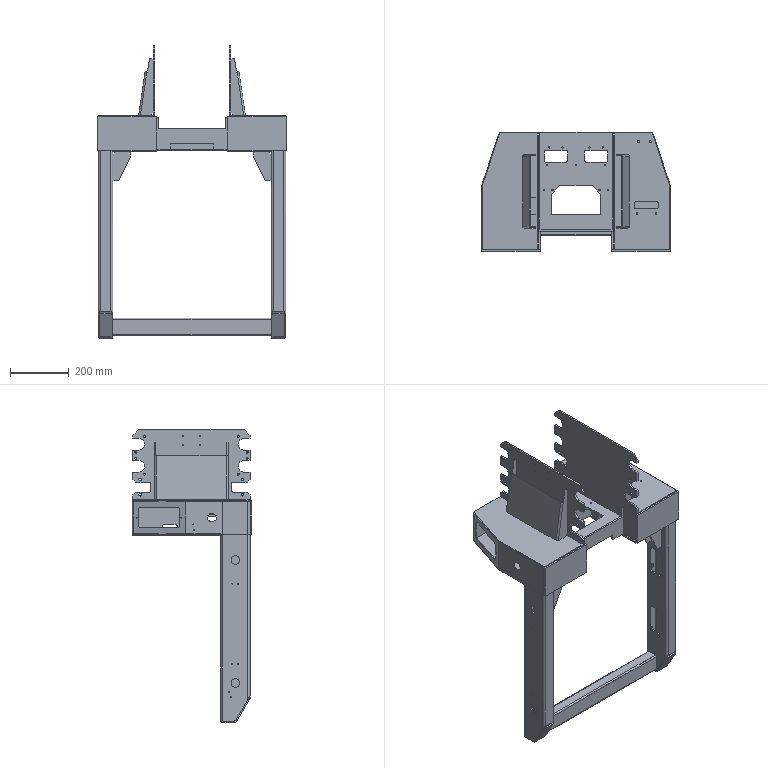Assembly | SolidWorks | mm | 23 component files | 23 solids | 730 faces | box 644 x 408 x 999 mm | volume 6835255 mm3 | plane 404 | cylinder 326 | commonest cylinder face diameters 3.3 x48 4.2 x46 20 x44 10 x37 6.8 x36 5 x20 9 x16 8 x16
Bill of materials:
JHK-B1001LeftRectangularTubeBeam | 1 | Q235A | Straight hollow rectangular tube with rounded corners. One end is cut at an angle across part of the section, and one wide face has two small features spaced along its length.
JHK-B1002RightRectangularTubeBeam | 1 | Q235A | Straight hollow rectangular tube with rounded corners and an angled cut at one end. One face has two round holes spaced along its length, plus a few very small marks.
JHK-B1003RightRearBaffle | 1 | Q235A | Flat plate of constant thickness, outline rectangular except for one long diagonal edge that trims a corner. It has a rounded-rectangle through slot and four small round holes.
JHK-B1004Stiffener | 4 | Q235A | Solid block extruded from a constant-thickness irregular quadrilateral profile: one straight vertical edge, a short chamfer at one top corner, and a long inclined edge that tapers the shape toward the bottom.
THK-B1001RollerBracketLeft | 1 | Q235A | Thin flat plate with a near-symmetric outline: chamfered top corners, two rounded U-shaped slots and one rectangular notch on each side edge, and rectangular notches plus a narrow slit along the bottom edge. It has multiple round holes, including a four-hole pattern near the top center.
THK-B1002RollerBracketRight | 1 | Q235A | Thin flat plate with chamfered top corners, paired U-shaped side slots, rectangular side notches, bottom-edge rectangular notches and a slit, and multiple round holes.
THK-B1003LeftRearBaffle | 1 | Q235A | Flat plate of constant thickness with one long diagonal edge trimming a corner and a single rounded-rectangle notch cut into one straight edge. No holes.
THK-B1005LeftFrontBaffle | 1 | Q235A | Flat plate of constant thickness with one long diagonal edge, a stepped rectangular cutout at one corner (L-shaped outline), and two small round holes along the straight edge.
THK-B1006RightFrontBaffle | 1 | Q235A | Flat plate of constant thickness with one long diagonal edge, a stepped rectangular corner cutout, a rounded-square through opening, two tiny holes above the opening, and two small holes along the straight edge.
THK-B1009MiddleSpacer | 1 | Q235A | Rectangular flat plate with small corner chamfers. It has two rounded-rectangle through openings, one large opening with chamfered upper corners, and many small round holes.
THK-B1011LooseRopeProtectionMountingPlate | 1 | Q235A | Rectangular flat bar with chamfered corners and two round through holes side by side near the center.
THK-B1012LowerBaffle | 1 | Q235A | Flat plate of constant thickness shaped as a long strip. Two narrow rectangular tabs project from the top edge near each end, and a wide shallow rectangular relief is cut into the middle of the bottom edge.
THK-B1013LowerSupportPlate | 2 | Q235A | Thin flat rectangular plate with uniform thickness and square edges; no holes or cutouts are visible.
THK-B1014SideStiffenerPlate | 2 | Q235A | Channel-shaped (C-section) formed part with a wide flat web and two side flanges joined by rounded bends. The flanges are tapered, so they are trapezoidal in side view, and they stick up past the web edge as narrow tabs. One bottom corner of each flange has a chamfer.
THK-B1015RectangularTubeEndSealingPlate | 2 | Q235A | Bent flat strip forming an angle shape: one longer leg slanted at an obtuse angle to a shorter flat leg, joined by a single rounded bend. The free-end corners are rounded and the thickness is uniform.
THK-B1016UpperCoverPlate | 1 | Q235A | Thin-wall formed band bracket, open at one side. It has a straight center segment, two angled segments and two parallel end legs. The top edge of the center segment has a wide rectangular notch. Each angled segment has a large rounded-rectangle cutout with small holes on either side of it. Each end leg has one round hole and a pair of small holes.
THK-B1017FrontCrossBeam | 1 | Q235A | Straight hollow rectangular tube with rounded outer and inner corners and constant wall thickness. Both ends are cut square and no holes are visible along its length.
Mates:
1. coincident | THK-B1003LeftRearBaffle-1 face at (-133, 200, -145) dir (0, 1, 0) | THK-B1005LeftFrontBaffle-1 face at (-260, 200, -255) dir (0, 1, 0)
2. coincident | JHK-B1003RightRearBaffle-1 face at (133, 200, -145) dir (0, 1, 0) | THK-B1006RightFrontBaffle-1 face at (122, 200, -255) dir (0, 1, 0)
3. coincident | THK-B1003LeftRearBaffle-1 face at (-133, 200, -145) dir (0, 1, 0) | JHK-B1003RightRearBaffle-1 face at (133, 200, -145) dir (0, 1, 0)
4. coincident | THK-B1003LeftRearBaffle-1 face at (-133, 200, -145) dir (0, 1, 0) | THK-B1016UpperCoverPlate-1 face at (-260, 200, -142) dir (0, -1, 0)
5. coincident | JHK-B1001LeftRectangularTubeBeam-1 plane at (-295, -150, -520) dir (0, 1, 0) | JHK-B1002RightRectangularTubeBeam-1 plane at (295, -150, -520) dir (0, 1, 0)
6. coincident | JHK-B1001LeftRectangularTubeBeam-1 plane at (-295, -150, -520) dir (0, 0, 1) | JHK-B1002RightRectangularTubeBeam-1 plane at (295, -150, -520) dir (0, 0, 1)
7. coincident | JHK-B1003RightRearBaffle-1 face at (226.5, 0, -145) dir (0, 0, -1) | JHK-B1002RightRectangularTubeBeam-1 face at (312.5, -192.5, -145) dir (0, 0, 1)
8. distance | JHK-B1002RightRectangularTubeBeam-1 face at (320, -192.5, -145) dir (1, 0, 0) | JHK-B1001LeftRectangularTubeBeam-1 face at (-320, -192.5, -145) dir (-1, 0, 0)
9. symmetric | JHK-B1001LeftRectangularTubeBeam-1 face at (-320, -192.5, -145) dir (-1, 0, 0) | JHK-B1002RightRectangularTubeBeam-1 face at (320, -192.5, -145) dir (1, 0, 0) | assembly plane at (0, 0, 0) dir (1, 0, 0)
10. coincident | THK-B1005LeftFrontBaffle-1 face at (-275, -100, -255) dir (0, -1, 0) | JHK-B1001LeftRectangularTubeBeam-1 face at (-277.5, -100, -145) dir (0, 1, 0)
11. coincident | THK-B1005LeftFrontBaffle-1 face at (-270, -200, -255) dir (-1, 0, 0) | JHK-B1001LeftRectangularTubeBeam-1 face at (-270, -192.5, -145) dir (1, 0, 0)
12. coincident | THK-B1006RightFrontBaffle-1 face at (270, -200, -255) dir (1, 0, 0) | JHK-B1002RightRectangularTubeBeam-1 face at (270, -192.5, -145) dir (-1, 0, 0)
13. coincident | THK-B1011LooseRopeProtectionMountingPlate-1 plane at (0, 23, -225) dir (1, 0, 0) | assembly plane at (0, 0, 0) dir (1, 0, 0)
14. coincident | THK-B1001RollerBracketLeft-1 plane at (-130, 0, 0) dir (0, 1, 0) | THK-B1002RollerBracketRight-1 plane at (130, 0, 0) dir (0, 1, 0)
15. distance | THK-B1001RollerBracketLeft-1 face at (-127, -179, -25) dir (1, 0, 0) | THK-B1002RollerBracketRight-1 face at (127, -179, -25) dir (-1, 0, 0)
16. symmetric | THK-B1001RollerBracketLeft-1 face at (-127, -179, -25) dir (1, 0, 0) | THK-B1002RollerBracketRight-1 face at (127, -179, -25) dir (-1, 0, 0) | assembly plane at (0, 0, 0) dir (1, 0, 0)
17. coincident | THK-B1006RightFrontBaffle-1 face at (273.5, -103.5, -255) dir (0, 0, 1) | THK-B1002RollerBracketRight-1 face at (127, 200, -255) dir (0, 0, -1)
18. coincident | THK-B1009MiddleSpacer-2 plane at (0, 36, -192) dir (1, 0, 0) | assembly plane at (0, 0, 0) dir (1, 0, 0)
19. coincident | THK-B1009MiddleSpacer-2 face at (55, 20, -195) dir (0, -1, 0) | THK-B1011LooseRopeProtectionMountingPlate-1 face at (0, 20, -225) dir (0, -1, 0)
20. coincident | THK-B1017FrontCrossBeam-2 plane at (0, -130, -860) dir (1, 0, 0) | assembly plane at (0, 0, 0) dir (1, 0, 0)
21. distance | JHK-B1001LeftRectangularTubeBeam-1 face at (-277.5, -100, -145) dir (0, 1, 0) | THK-B1017FrontCrossBeam-2 face at (270, -110, -835) dir (0, 1, 0)
22. coincident | JHK-B1001LeftRectangularTubeBeam-1 face at (-277.5, -192.5, -895) dir (0, 0, -1) | THK-B1015RectangularTubeEndSealingPlate-1 face at (-273, -102, -895) dir (0, 0, 1)
23. coincident | JHK-B1001LeftRectangularTubeBeam-1 plane at (-295, -150, -520) dir (1, 0, 0) | THK-B1015RectangularTubeEndSealingPlate-1 plane at (-295, -150, -895) dir (1, 0, 0)
24. distance | JHK-B1001LeftRectangularTubeBeam-1 face at (-277.5, -192.5, -895) dir (0, 0, -1) | THK-B1017FrontCrossBeam-2 face at (270, -145, -890) dir (0, 0, -1)
25. coincident | THK-B1009MiddleSpacer-2 face at (0, 36, -195) dir (0, 0, -1) | THK-B1011LooseRopeProtectionMountingPlate-1 face at (-126, 26, -195) dir (0, 0, 1)
26. distance | JHK-B1001LeftRectangularTubeBeam-1 face at (-312.5, -105, -145) dir (0, -1, 0) | THK-B1015RectangularTubeEndSealingPlate-1 face at (-273, -102, -895) dir (0, 1, 0)
27. coincident | THK-B1015RectangularTubeEndSealingPlate-1 face at (-273, -102, -899) dir (0, 0, -1) | THK-B1015RectangularTubeEndSealingPlate-2 face at (317, -102, -899) dir (0, 0, -1)
28. coincident | THK-B1015RectangularTubeEndSealingPlate-1 face at (-273, -102, -895) dir (0, 1, 0) | THK-B1015RectangularTubeEndSealingPlate-2 face at (317, -102, -895) dir (0, 1, 0)
29. coincident | JHK-B1002RightRectangularTubeBeam-1 plane at (295, -150, -520) dir (1, 0, 0) | THK-B1015RectangularTubeEndSealingPlate-2 plane at (295, -150, -895) dir (1, 0, 0)
30. coincident | THK-B1003LeftRearBaffle-1 face at (-133, -200, -145) dir (1, 0, 0) | THK-B1001RollerBracketLeft-1 face at (-133, -179, -25) dir (-1, 0, 0)
31. coincident | THK-B1002RollerBracketRight-1 face at (133, -179, -25) dir (1, 0, 0) | JHK-B1003RightRearBaffle-1 face at (133, 200, -145) dir (-1, 0, 0)
32. coincident | THK-B1001RollerBracketLeft-1 plane at (-130, 0, 0) dir (0, 0, -1) | THK-B1002RollerBracketRight-1 plane at (130, 0, 0) dir (0, 0, -1)
33. coincident | THK-B1001RollerBracketLeft-1 plane at (-130, 0, 0) dir (0, 0, -1) | assembly plane at (0, 0, 0) dir (0, 0, 1)
34. coincident | THK-B1001RollerBracketLeft-1 plane at (-130, 0, 0) dir (0, 1, 0) | assembly plane at (0, 0, 0) dir (0, 1, 0)
35. symmetric | THK-B1001RollerBracketLeft-1 plane at (-130, 0, 0) dir (-1, 0, 0) | THK-B1002RollerBracketRight-1 plane at (130, 0, 0) dir (-1, 0, 0) | assembly plane at (0, 0, 0) dir (1, 0, 0)
36. distance | THK-B1006RightFrontBaffle-1 face at (273.5, -103.5, -255) dir (0, 0, 1) | JHK-B1003RightRearBaffle-1 face at (226.5, 0, -145) dir (0, 0, -1)
37. coincident | THK-B1005LeftFrontBaffle-1 face at (-275, -105, -261) dir (0, 0, -1) | THK-B1006RightFrontBaffle-1 face at (273.5, -103.5, -261) dir (0, 0, -1)
38. coincident | THK-B1003LeftRearBaffle-1 face at (-226.5, 0, -139) dir (0, 0, 1) | JHK-B1003RightRearBaffle-1 face at (226.5, 0, -139) dir (0, 0, 1)
39. coincident | THK-B1016UpperCoverPlate-1 plane at (0, 200, -200) dir (1, 0, 0) | assembly plane at (0, 0, 0) dir (1, 0, 0)
40. coincident | THK-B1001RollerBracketLeft-1 face at (-133, 200, -255) dir (0, 1, 0) | THK-B1016UpperCoverPlate-1 face at (-260, 200, -142) dir (0, -1, 0)
41. coincident | THK-B1016UpperCoverPlate-1 face at (-260, 202, -142) dir (0, 1, 0) | THK-B1009MiddleSpacer-2 face at (-126, 202, -189) dir (0, 1, 0)
42. distance | THK-B1009MiddleSpacer-2 face at (0, 36, -189) dir (0, 0, 1) | THK-B1003LeftRearBaffle-1 face at (-226.5, 0, -139) dir (0, 0, 1)
43. coincident | JHK-B1001LeftRectangularTubeBeam-1 face at (-277.5, -200, -145) dir (0, -1, 0) | THK-B1013LowerSupportPlate-3 face at (-222, -200, -200) dir (0, 1, 0)
44. coincident | JHK-B1002RightRectangularTubeBeam-1 face at (312.5, -200, -145) dir (0, -1, 0) | THK-B1013LowerSupportPlate-4 face at (222, -200, -200) dir (0, 1, 0)
45. coincident | THK-B1012LowerBaffle-1 plane at (0, -130, -200) dir (1, 0, 0) | assembly plane at (0, 0, 0) dir (1, 0, 0)
46. coincident | THK-B1001RollerBracketLeft-1 face at (-133, -136, -182) dir (0, 1, 0) | THK-B1012LowerBaffle-1 face at (-140, -136, -145) dir (0, -1, 0)
47. coincident | THK-B1001RollerBracketLeft-1 face at (-133, -136, -255) dir (0, 0, -1) | THK-B1012LowerBaffle-1 face at (0, -130, -255) dir (0, 0, -1)
48. coincident | THK-B1013LowerSupportPlate-3 plane at (-222, -203, -200) dir (0, 0, 1) | THK-B1013LowerSupportPlate-4 plane at (222, -203, -200) dir (0, 0, 1)
49. symmetric | THK-B1013LowerSupportPlate-3 plane at (-222, -203, -200) dir (1, 0, 0) | THK-B1013LowerSupportPlate-4 plane at (222, -203, -200) dir (1, 0, 0) | assembly plane at (0, 0, 0) dir (1, 0, 0)
50. distance | THK-B1001RollerBracketLeft-1 face at (-127, -179, -25) dir (1, 0, 0) | THK-B1013LowerSupportPlate-3 face at (-122, -200, -142) dir (1, 0, 0)
51. width | THK-B1006RightFrontBaffle-1 face at (273.5, -103.5, -261) dir (0, 0, -1) | JHK-B1003RightRearBaffle-1 face at (226.5, 0, -139) dir (0, 0, 1) | THK-B1016UpperCoverPlate-1 face at (262.581, 198.581, -142) dir (0, 0, 1) | THK-B1016UpperCoverPlate-1 face at (-262.581, 198.581, -258) dir (0, 0, -1)
52. coincident | THK-B1014SideStiffenerPlate-3 plane at (167.613, 0, -40.205) dir (0, -1, 0) | assembly plane at (0, 0, 0) dir (0, 1, 0)
53. coincident | THK-B1002RollerBracketRight-1 face at (133, -179, -25) dir (1, 0, 0) | THK-B1014SideStiffenerPlate-3 face at (133, 121, -139.099) dir (-1, 0, 0)
54. coincident | JHK-B1003RightRearBaffle-1 face at (226.5, 0, -139) dir (0, 0, 1) | THK-B1014SideStiffenerPlate-3 face at (176.365, 125, -139) dir (0, 0, -1)
55. coincident | THK-B1001RollerBracketLeft-1 face at (-133, -179, -25) dir (-1, 0, 0) | THK-B1014SideStiffenerPlate-4 face at (-133, 121, -146.516) dir (1, 0, 0)
56. coincident | THK-B1003LeftRearBaffle-1 face at (-226.5, 0, -139) dir (0, 0, 1) | THK-B1014SideStiffenerPlate-4 face at (-176.365, -125, -139) dir (0, 0, -1)
57. coincident | THK-B1014SideStiffenerPlate-3 plane at (167.613, 0, -40.205) dir (0, -1, 0) | THK-B1014SideStiffenerPlate-4 plane at (-167.613, 0, -40.205) dir (0, 1, 0)
58. width | THK-B1003LeftRearBaffle-1 face at (-226.5, 0, -139) dir (0, 0, 1) | THK-B1005LeftFrontBaffle-1 face at (-275, -105, -261) dir (0, 0, -1) | THK-B1013LowerSupportPlate-3 face at (-322, -200, -258) dir (0, 0, -1) | THK-B1013LowerSupportPlate-3 face at (-322, -200, -142) dir (0, 0, 1)
59. coincident | JHK-B1001LeftRectangularTubeBeam-1 face at (-270, -192.5, -145) dir (1, 0, 0) | JHK-B1004Stiffener-1 face at (-270, -178, -261) dir (-1, 0, 0)
60. coincident | THK-B1005LeftFrontBaffle-1 face at (-275, -105, -261) dir (0, 0, -1) | JHK-B1004Stiffener-1 face at (-210, -178, -261) dir (0, 0, 1)
61. coincident | JHK-B1004Stiffener-1 plane at (-270, -175, -261) dir (0, 0, 1) | JHK-B1004Stiffener-2 plane at (-270, -125, -261) dir (0, 0, 1)
62. coincident | JHK-B1004Stiffener-1 plane at (-270, -175, -261) dir (-1, 0, 0) | JHK-B1004Stiffener-2 plane at (-270, -125, -261) dir (-1, 0, 0)
63. distance | JHK-B1004Stiffener-1 plane at (-270, -175, -261) dir (0, -1, 0) | JHK-B1004Stiffener-2 plane at (-270, -125, -261) dir (0, -1, 0)
64. width | JHK-B1001LeftRectangularTubeBeam-1 face at (-277.5, -100, -145) dir (0, 1, 0) | JHK-B1001LeftRectangularTubeBeam-1 face at (-277.5, -200, -145) dir (0, -1, 0) | JHK-B1004Stiffener-1 face at (-270, -178, -261) dir (0, -1, 0) | JHK-B1004Stiffener-2 face at (-270, -122, -261) dir (0, 1, 0)
65. coincident | JHK-B1004Stiffener-1 plane at (-270, -175, -261) dir (0, 0, 1) | JHK-B1004Stiffener-3 plane at (270, -125, -261) dir (0, 0, 1)
66. coincident | JHK-B1004Stiffener-1 plane at (-270, -175, -261) dir (0, -1, 0) | JHK-B1004Stiffener-4 plane at (270, -175, -261) dir (0, 1, 0)
67. coincident | JHK-B1004Stiffener-2 plane at (-270, -125, -261) dir (0, -1, 0) | JHK-B1004Stiffener-3 plane at (270, -125, -261) dir (0, 1, 0)
68. coincident | JHK-B1004Stiffener-3 plane at (270, -125, -261) dir (0, 0, 1) | JHK-B1004Stiffener-4 plane at (270, -175, -261) dir (0, 0, 1)
69. coincident | JHK-B1004Stiffener-3 plane at (270, -125, -261) dir (1, 0, 0) | JHK-B1004Stiffener-4 plane at (270, -175, -261) dir (1, 0, 0)
70. coincident | JHK-B1002RightRectangularTubeBeam-1 face at (270, -192.5, -145) dir (-1, 0, 0) | JHK-B1004Stiffener-3 face at (270, -122, -261) dir (1, 0, 0)